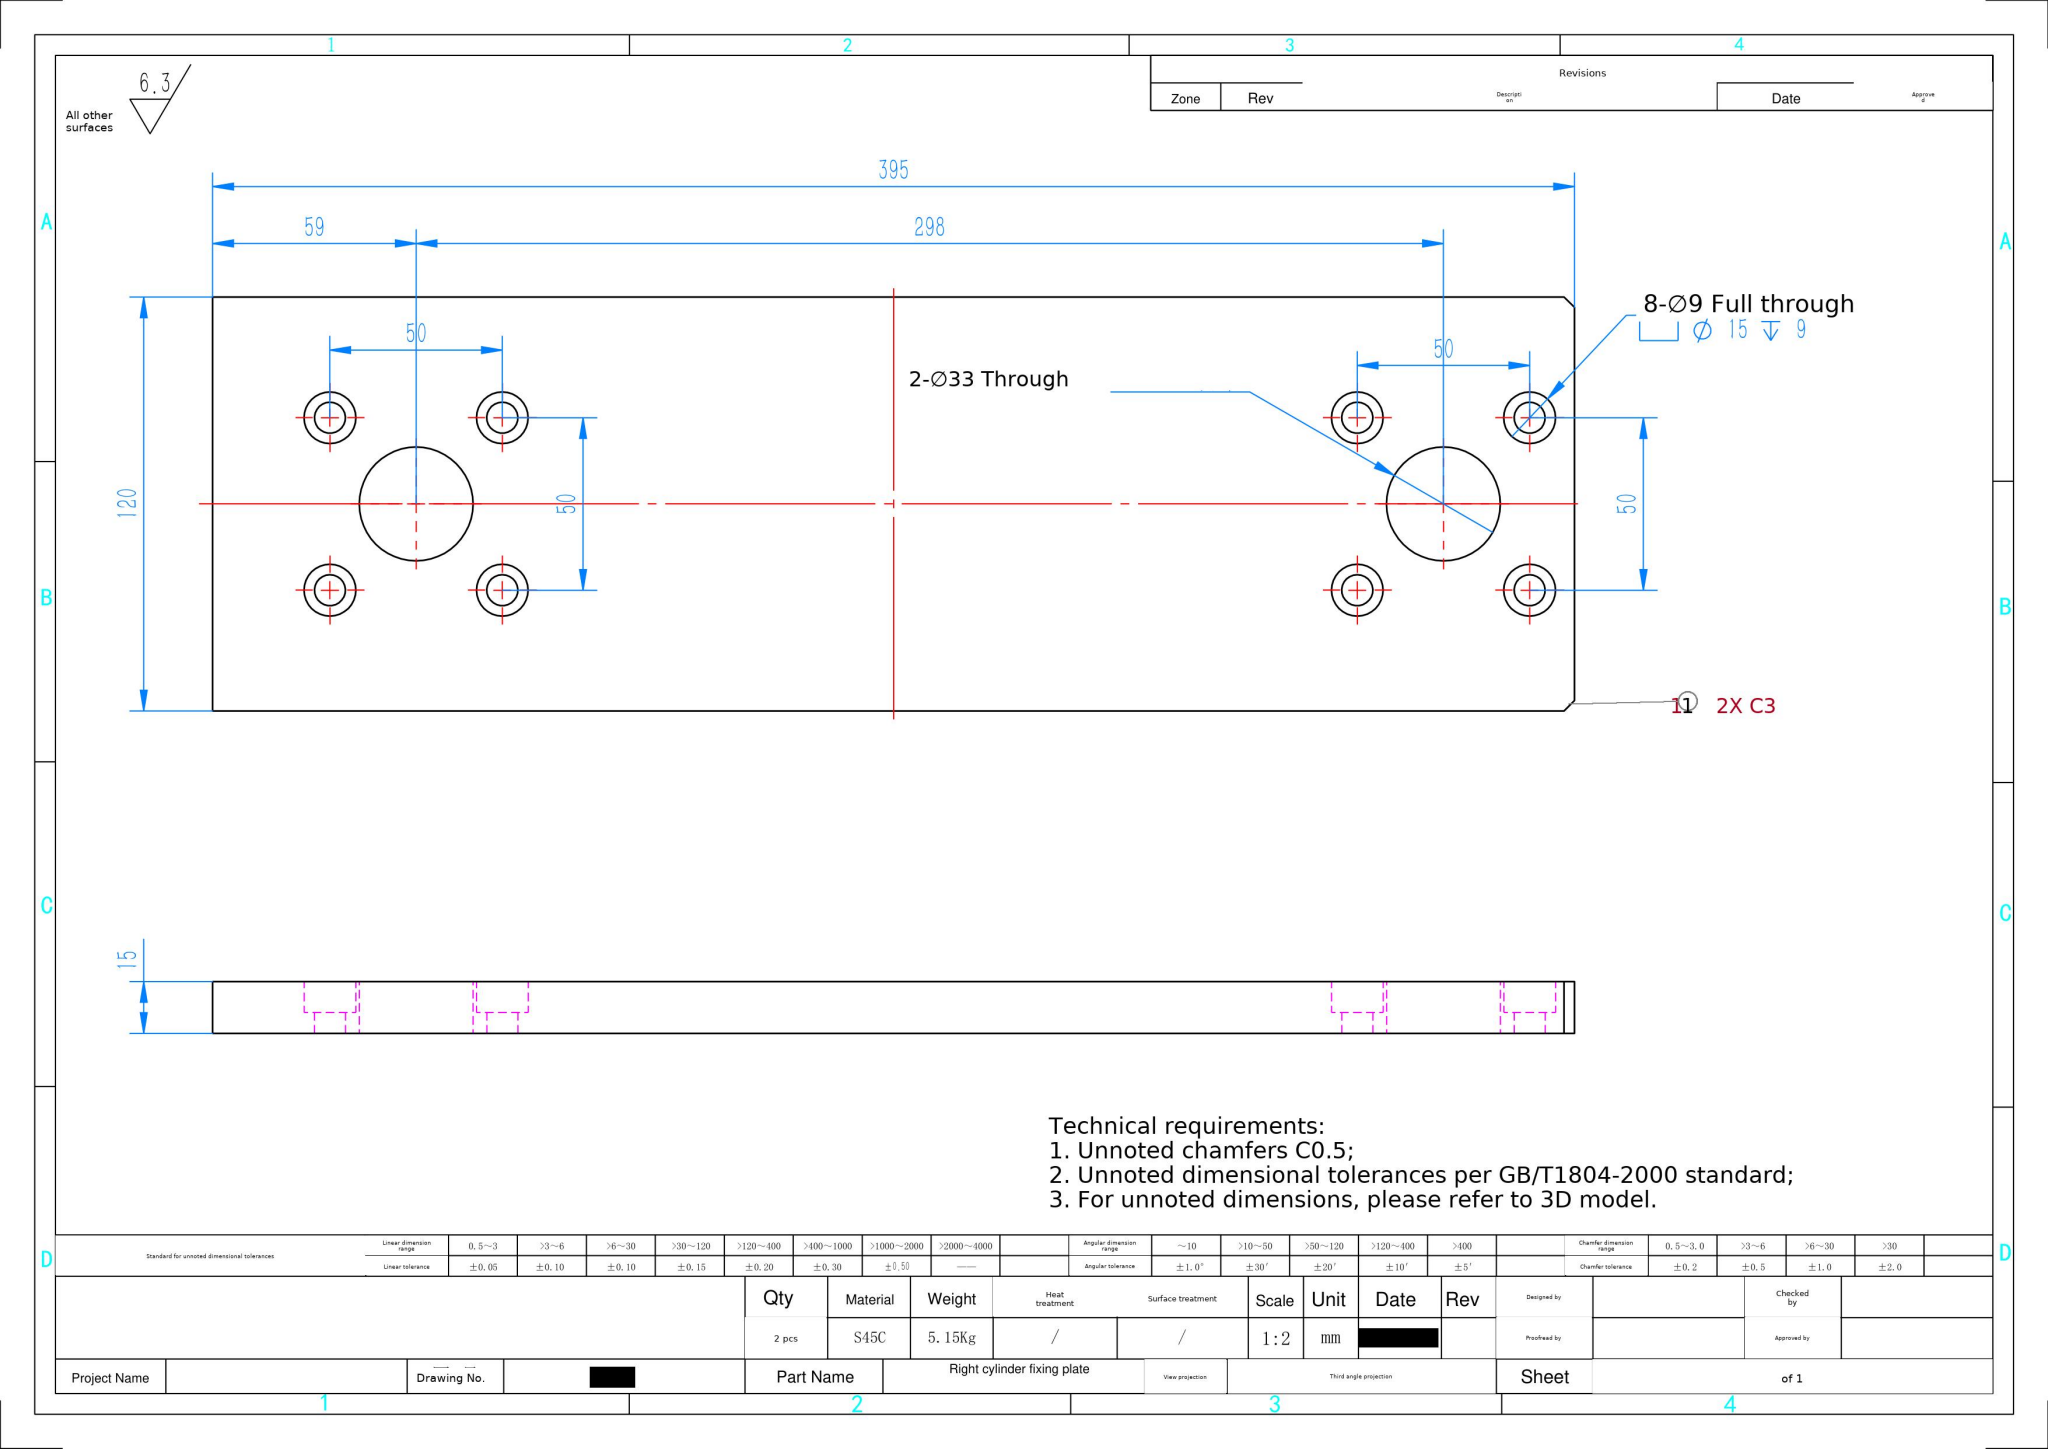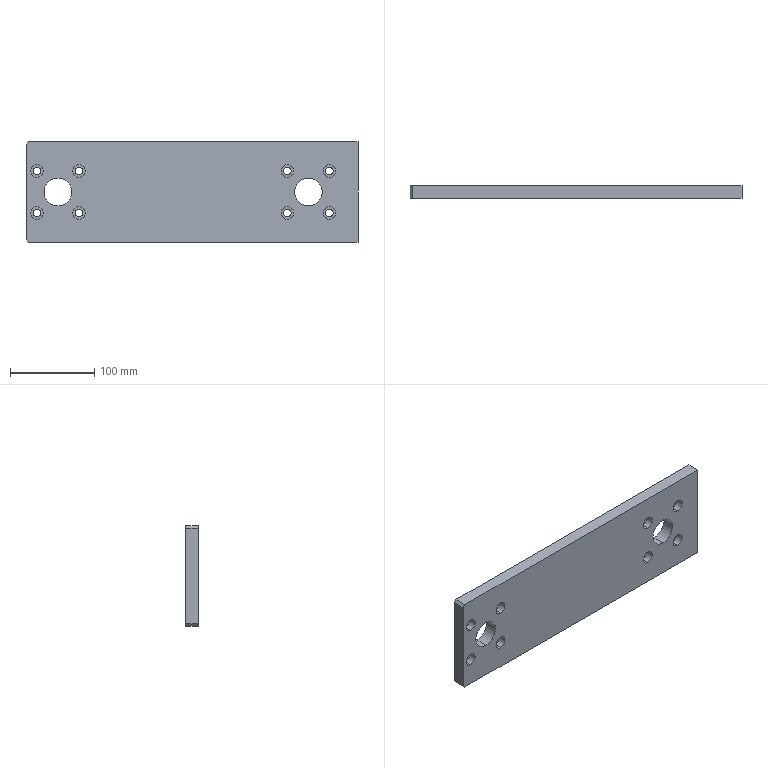Part | SolidWorks | mm | material S45C | 1 solid | 52 faces | box 395 x 15 x 120 mm | volume 669429 mm3 | cylinder 36 | plane 16 | commonest cylinder face diameters 15 x16 9 x16 33 x4
build123d program:
from build123d import *

# Parameters (mm, degrees)
SKETCH1_W                                       = 395
SKETCH1_H                                       = 120
BOSS_EXTRUDE1_DEPTH                             = 15
SKETCH2_R                                       = 16.5
CUT_EXTRUDE1_DEPTH                              = 207.957
M8_HEX_SOCKET_HEAD_CAP_SCREW_CBORE1_D           = 9
M8_HEX_SOCKET_HEAD_CAP_SCREW_CBORE1_CBORE_D     = 15
M8_HEX_SOCKET_HEAD_CAP_SCREW_CBORE1_CBORE_DEPTH = 9
CHAMFER1_SIZE                                   = 3


with BuildPart() as part:
    # Sketch1 → Boss-Extrude1 (new body)
    with BuildSketch(Plane(origin=(0, 0, 0), x_dir=(1, 0, 0), z_dir=(0, 1, 0))):
        Rectangle(SKETCH1_W, SKETCH1_H)
    extrude(amount=BOSS_EXTRUDE1_DEPTH)

    # Sketch2 → Cut-Extrude1 (cut, through all)
    with BuildSketch(Plane.XZ):
        with Locations(Location((-159.5, 0, 0), (0, 0, 270))):
            Circle(SKETCH2_R)
        with Locations(Location((138.5, 0, 0), (0, 0, 90))):
            Circle(SKETCH2_R)
    extrude(amount=-CUT_EXTRUDE1_DEPTH, mode=Mode.SUBTRACT)

    # M8 Hex Socket Head Cap Screw CBORE1 (through all)
    with Locations(Plane.XZ):
        with Locations((-134.5, 25), (-184.5, -25), (-134.5, -25), (-184.5, 25), (163.5, 25), (113.5, -25), (163.5, -25), (113.5, 25)):
            CounterBoreHole(M8_HEX_SOCKET_HEAD_CAP_SCREW_CBORE1_D / 2, M8_HEX_SOCKET_HEAD_CAP_SCREW_CBORE1_CBORE_D / 2, M8_HEX_SOCKET_HEAD_CAP_SCREW_CBORE1_CBORE_DEPTH)

    # Chamfer1
    chamfer1_edges = [part.edges().sort_by_distance(p)[0] for p in [
        (-197.5, 7.5, 60),
        (-197.5, 7.5, -60),
    ]]
    chamfer(chamfer1_edges, length=CHAMFER1_SIZE)


solid = part.part